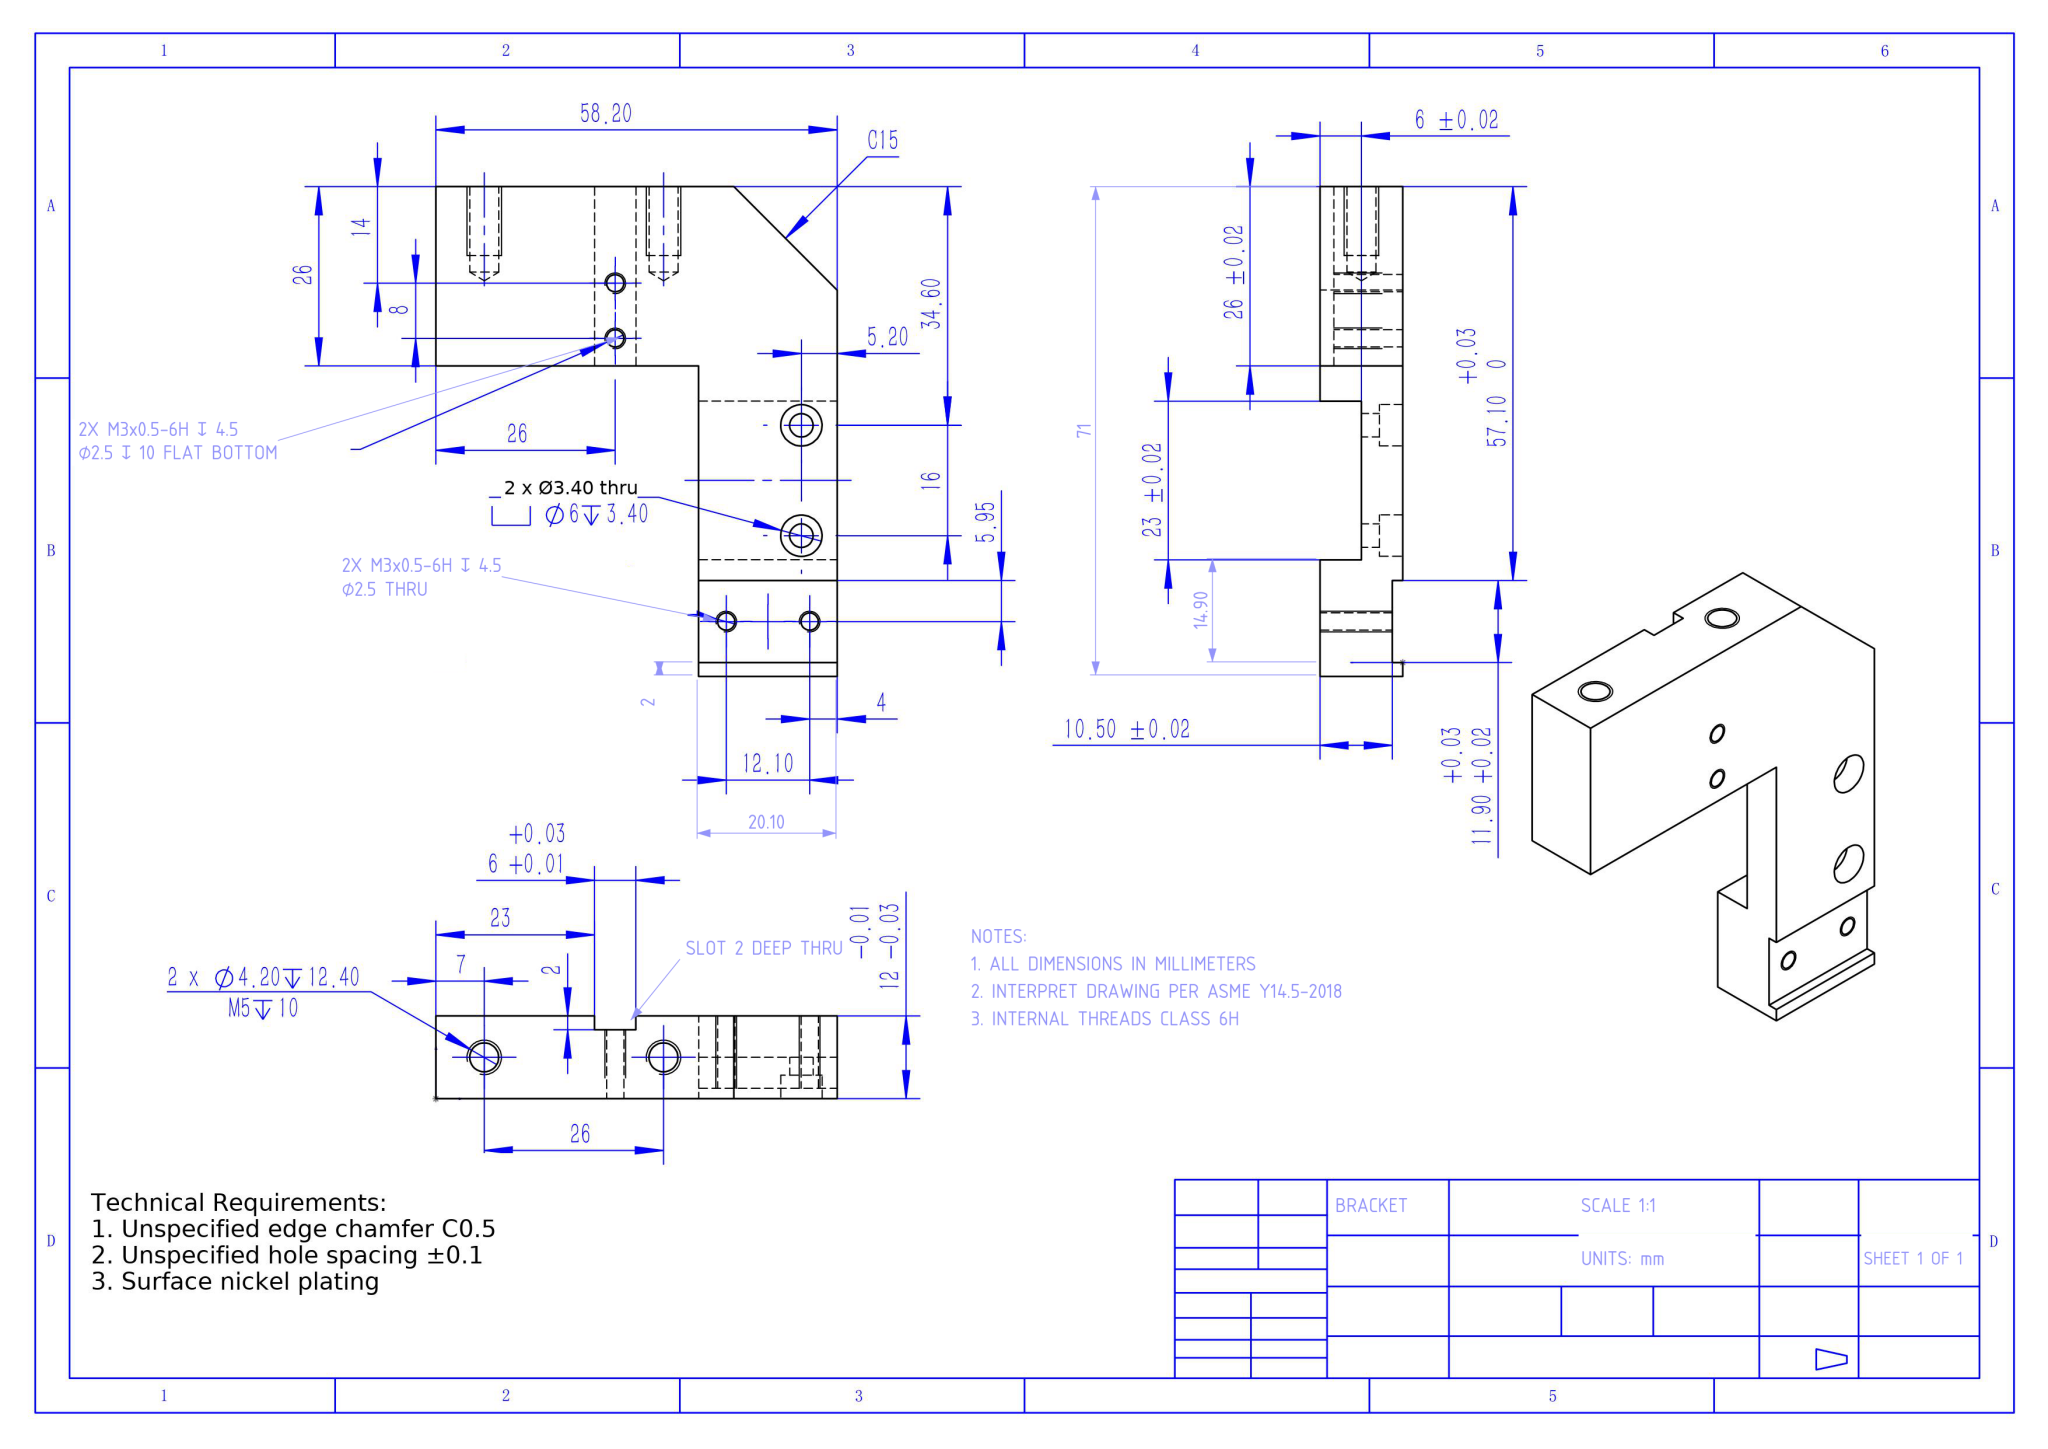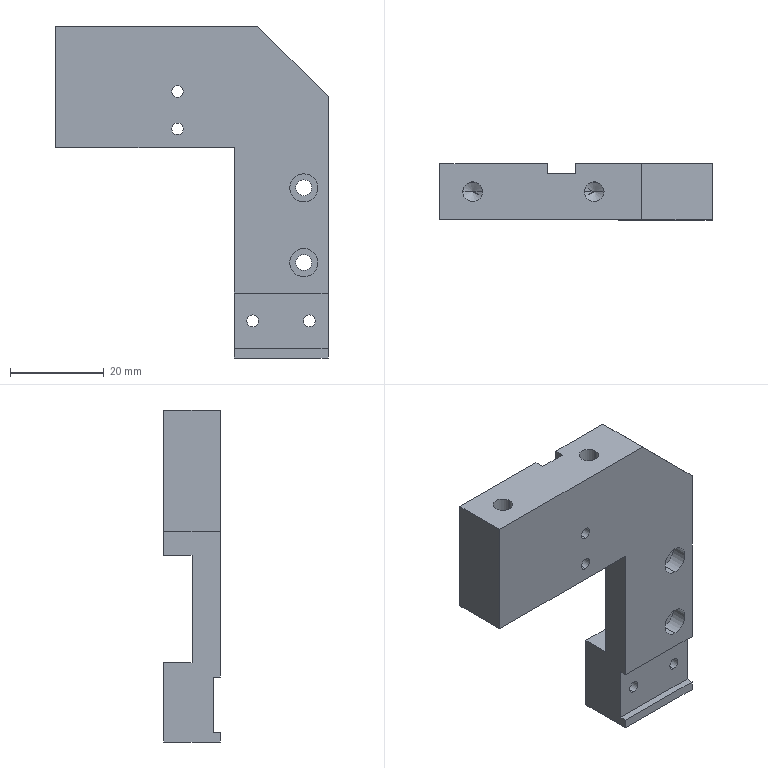Part | NX | mm | 1 solid | 47 faces | box 58.2 x 12 x 71 mm | volume 23422 mm3 | plane 23 | cylinder 20 | cone 4 | commonest cylinder face diameters 2.5 x8 6 x4 3.4 x4 4.2 x4